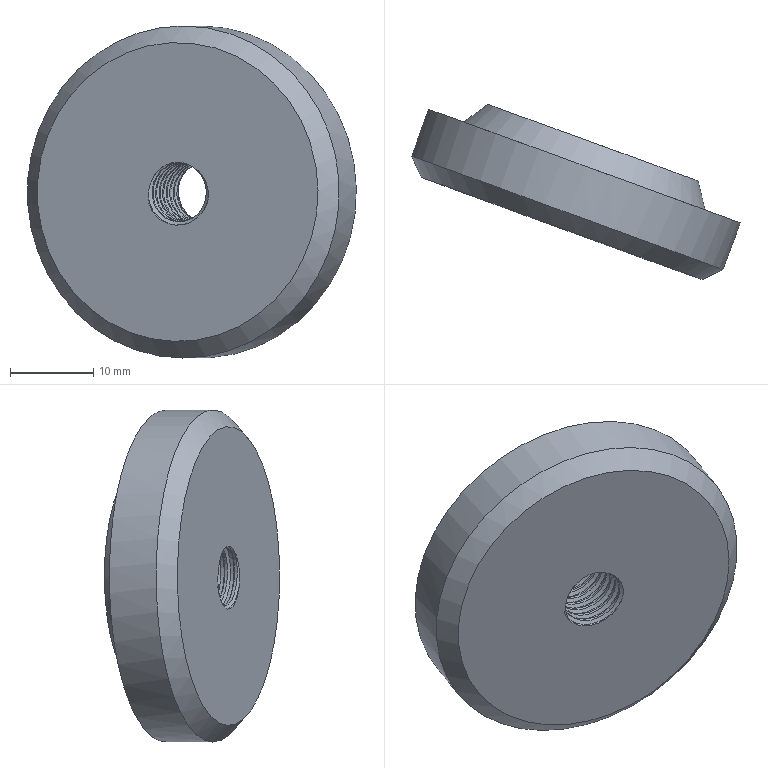Component | NX | 5 | 1 solid | 11 faces | volume 11293 mm3 | plane 3 | cone 3 | cylinder 3 | spline 2 | commonest cylinder face diameters 40 x1 7.188 x1 8 x1